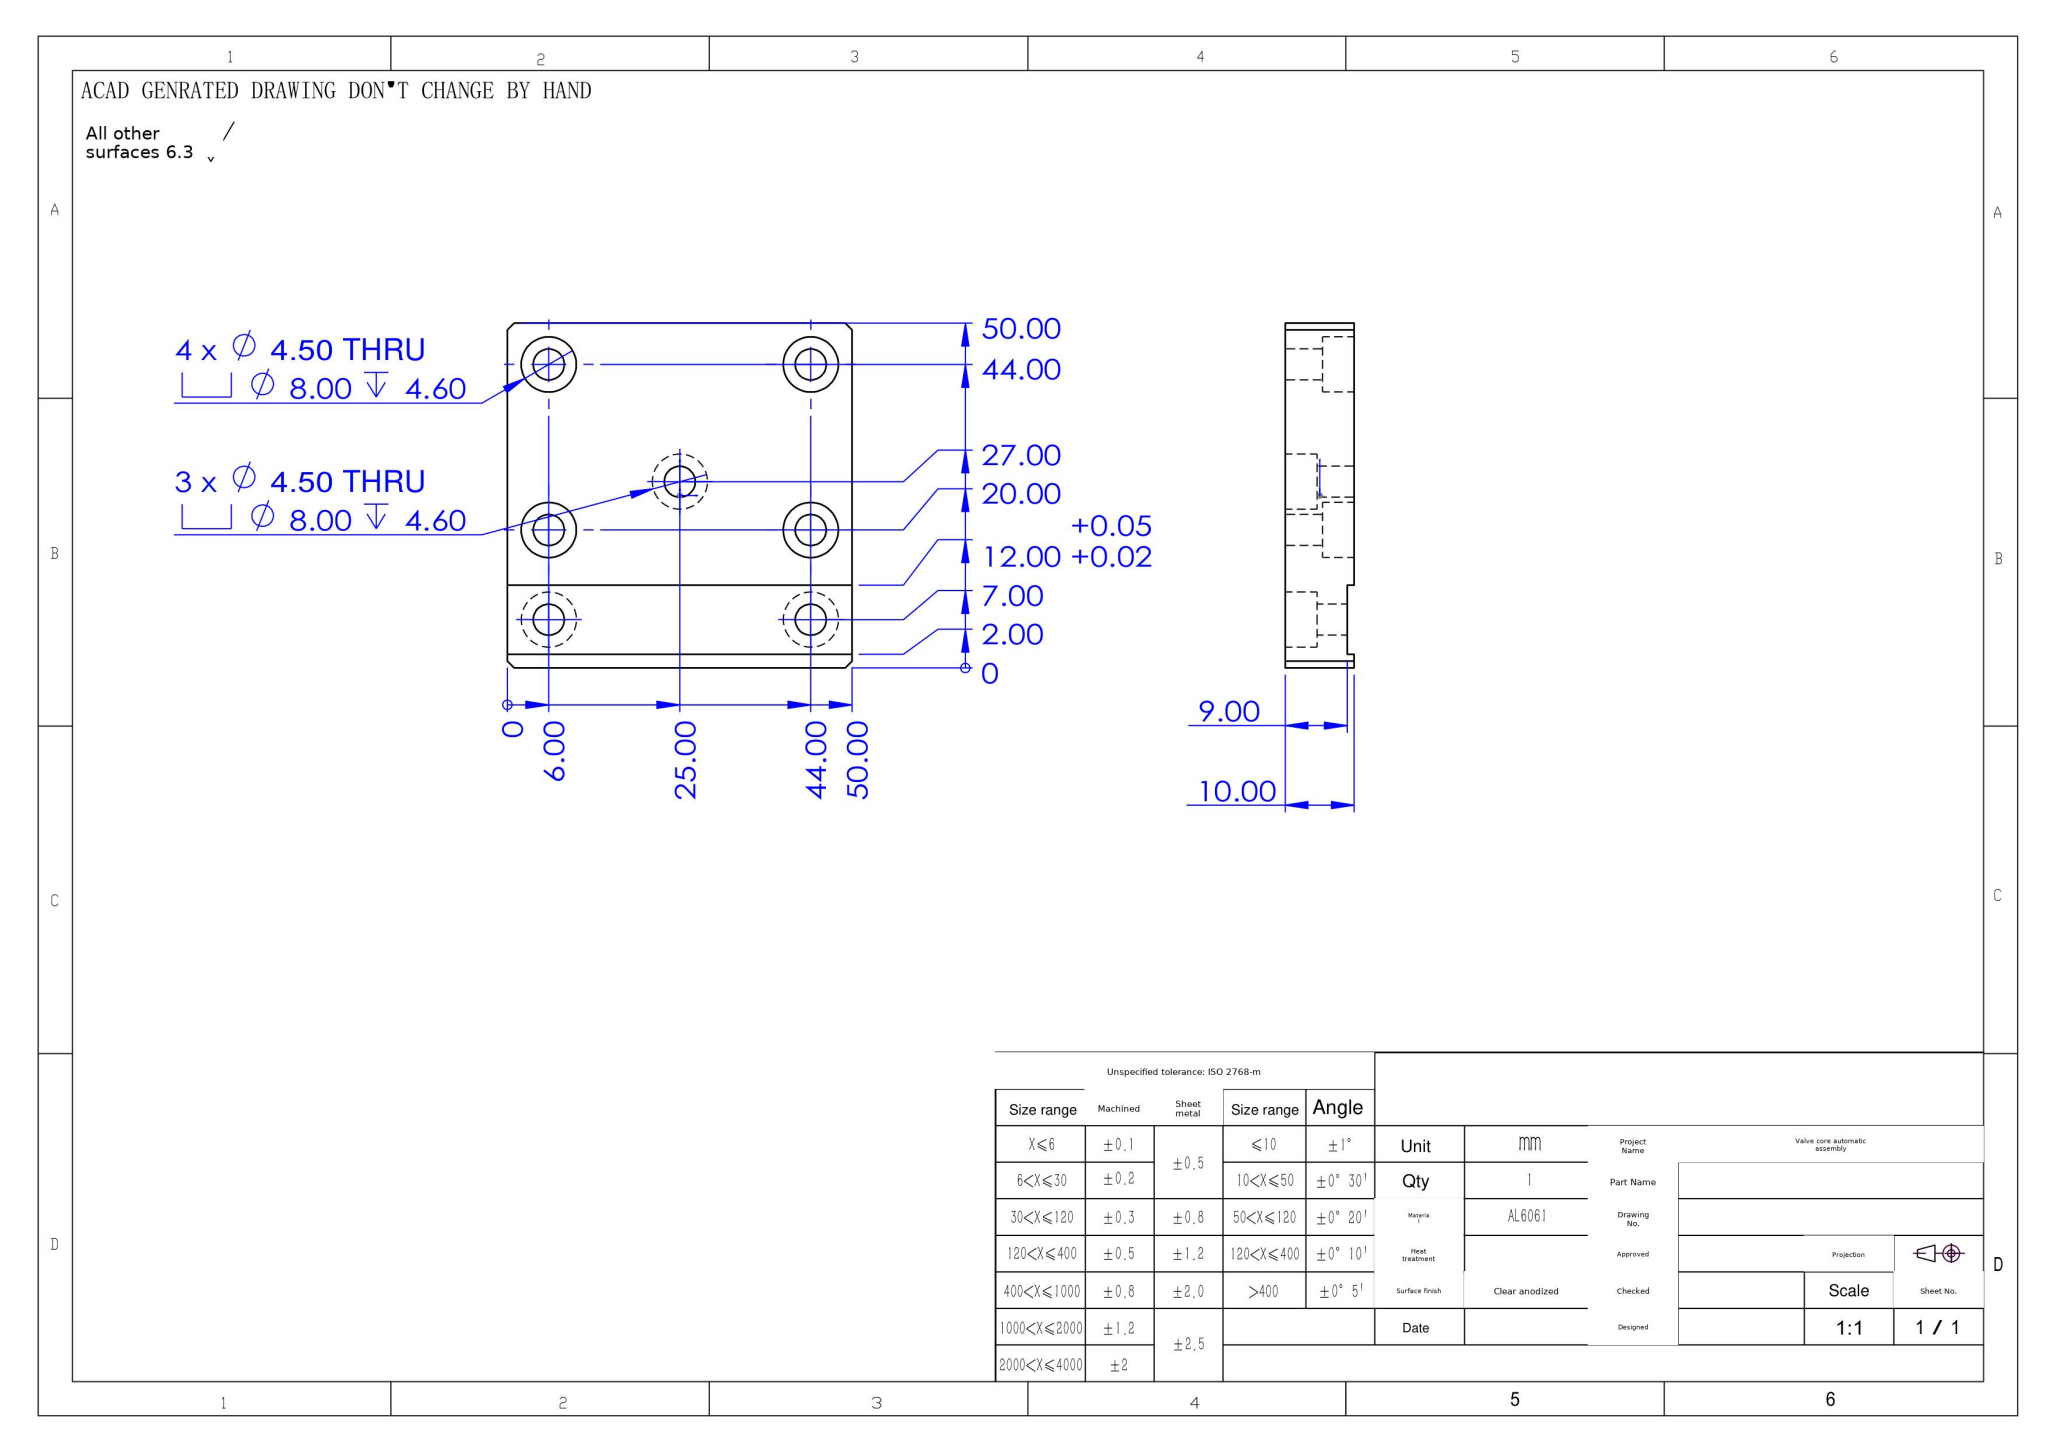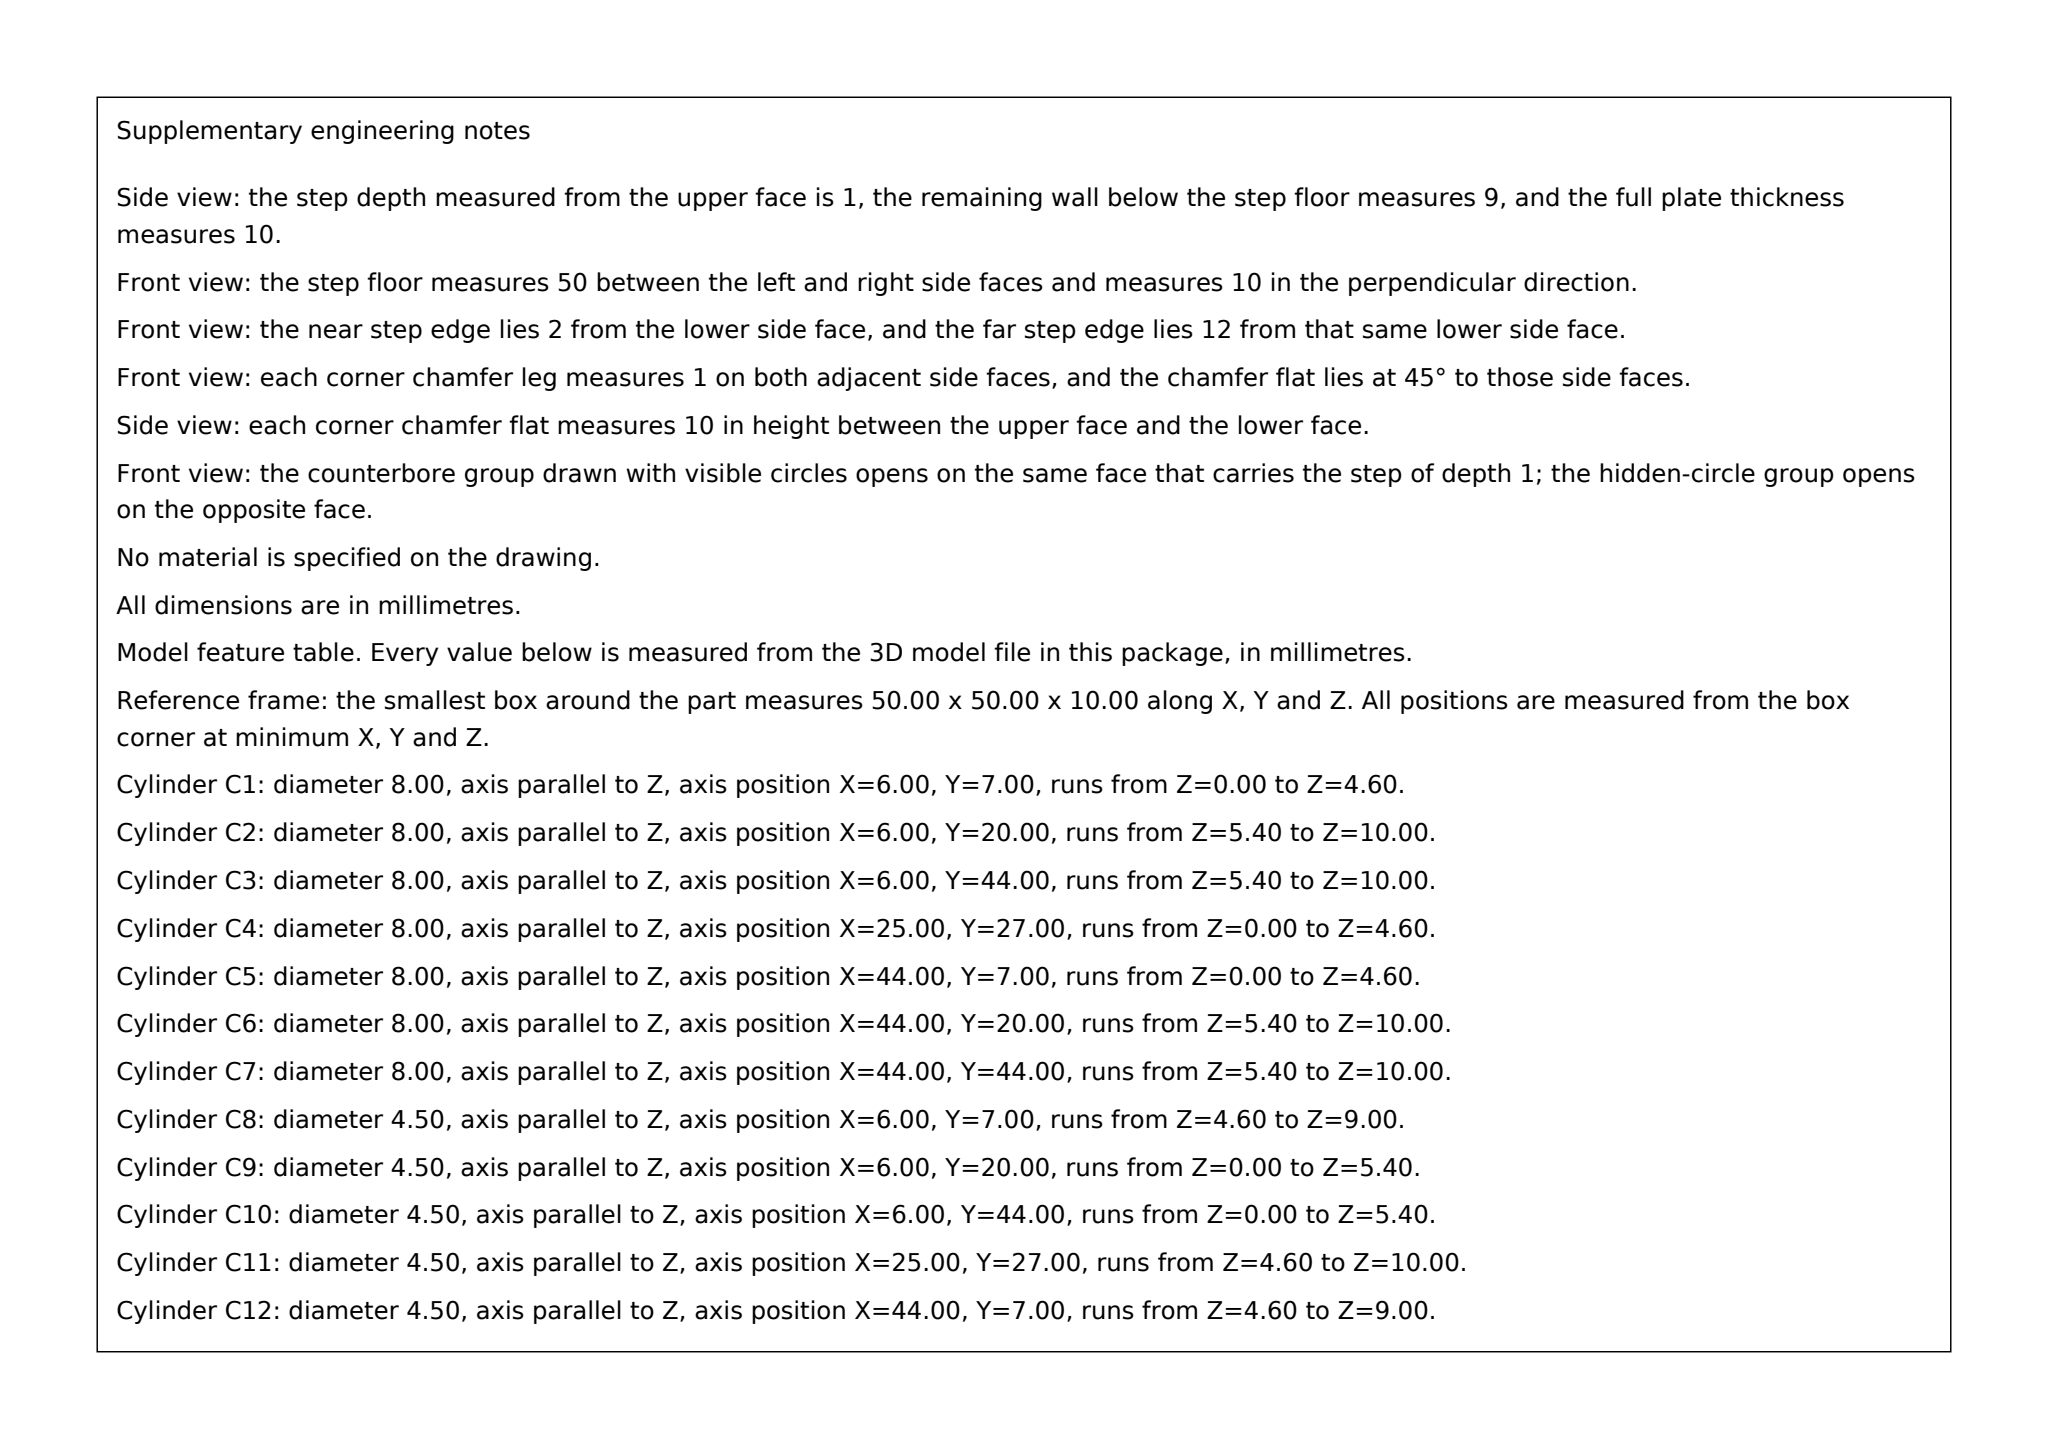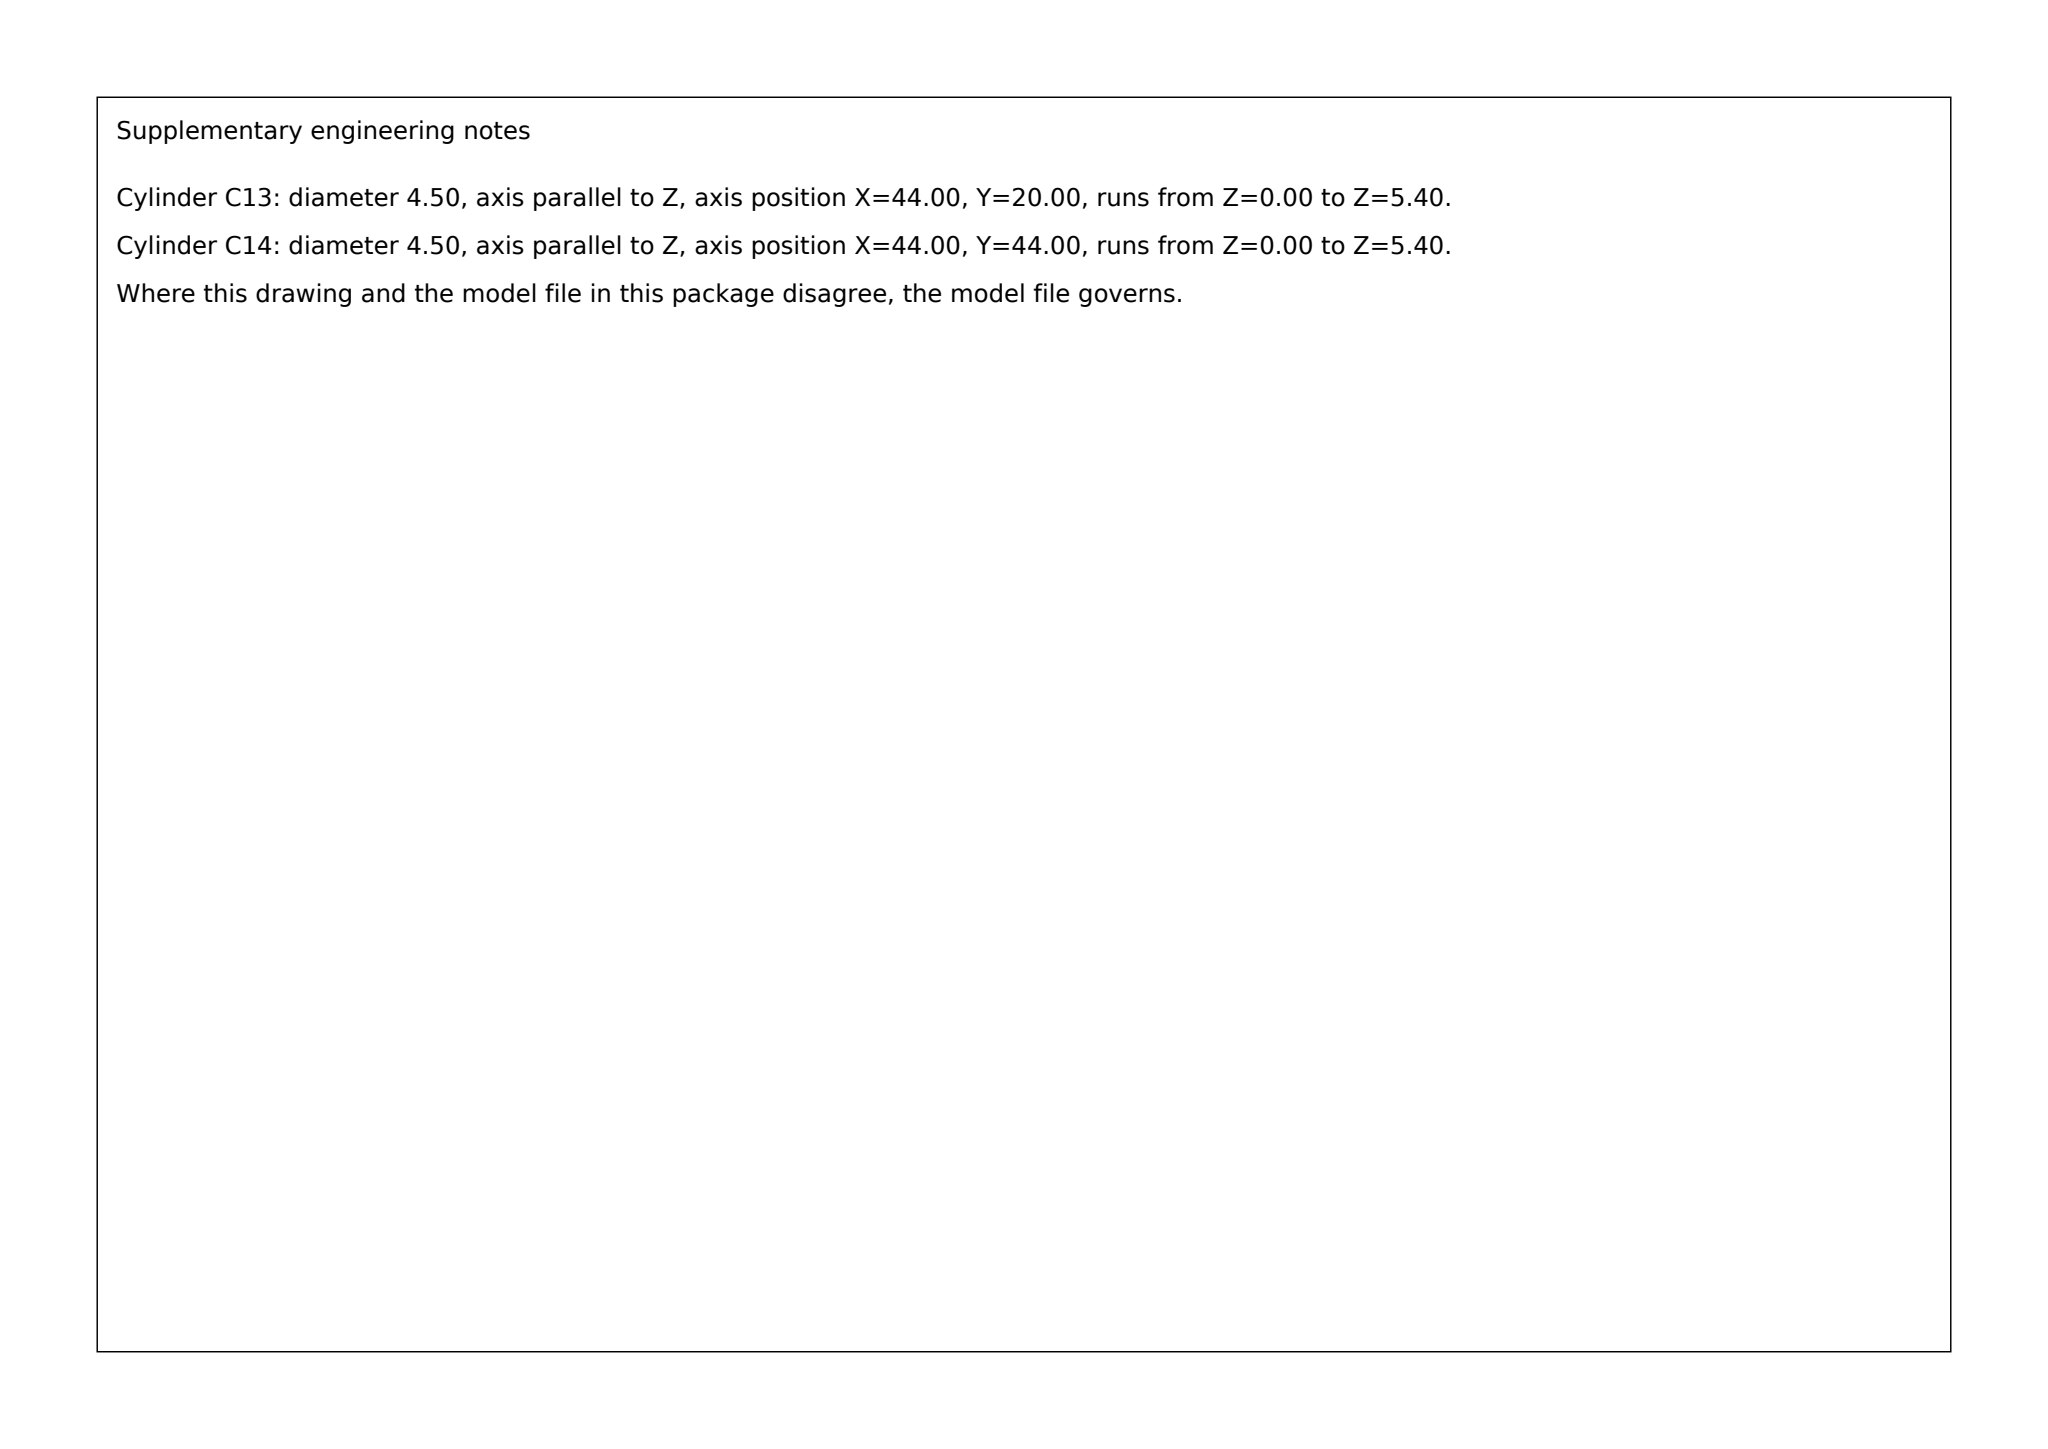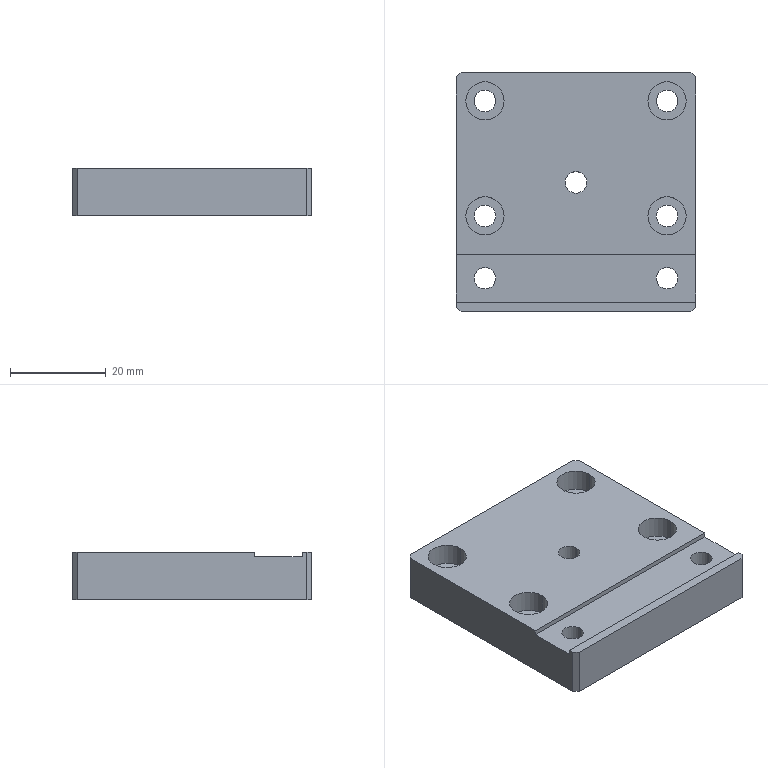Part | SolidWorks | mm | material AL6061 | 1 solid | 49 faces | box 50 x 50 x 10 mm | volume 22292 mm3 | cylinder 28 | plane 21 | commonest cylinder face diameters 8 x14 4.5 x14
Drawing notes:
STEP FACE 12.00 +0.05/+0.02 FROM BOTTOM EDGE (12.02-12.05) | from the solid: Plane normal y at offset 12.0 (x 0-50, z 9-10) bounding the 1 mm deep ledge; measured from y=0 face, datum used by the 2.00/7.00/20.00/27.00/44.00/50.00 vertical chain
build123d program:
from build123d import *

# Parameters (mm, degrees)
SKETCH1_W                                          = 50
SKETCH1_H                                          = 50
BOSS_EXTRUDE1_DEPTH                                = 5
SKETCH2_W                                          = 50
SKETCH2_H                                          = 10
CUT_EXTRUDE1_DEPTH                                 = 1
HOLE_SIZE_ACCORDING_TO_TYPE_1_OF_HEXAG_D           = 4.5
HOLE_SIZE_ACCORDING_TO_TYPE_1_OF_HEXAG_CBORE_D     = 8
HOLE_SIZE_ACCORDING_TO_TYPE_1_OF_HEXAG_CBORE_DEPTH = 4.6
HOLE_SIZE_ACCORDING_TO_TYPE_2_OF_HEXAG_D           = 4.5
HOLE_SIZE_ACCORDING_TO_TYPE_2_OF_HEXAG_CBORE_D     = 8
HOLE_SIZE_ACCORDING_TO_TYPE_2_OF_HEXAG_CBORE_DEPTH = 4.6
CHAMFER1_SIZE                                      = 1


with BuildPart() as part:
    # Sketch1 → Boss-Extrude1 (new, symmetric)
    with BuildSketch(Plane.XY):
        Rectangle(SKETCH1_W, SKETCH1_H)
    extrude(amount=BOSS_EXTRUDE1_DEPTH, both=True)

    # Sketch2 → Cut-Extrude1 (cut)
    with BuildSketch(Plane.XY.offset(5)):
        with Locations((0, -18)):
            Rectangle(SKETCH2_W, SKETCH2_H)
    extrude(amount=-CUT_EXTRUDE1_DEPTH, mode=Mode.SUBTRACT)

    # Hole Size _According to_ Type 1 of Hexag (through all)
    with Locations(Plane(origin=(0, 0, -5), x_dir=(-1, 0, 0), z_dir=(0, 0, -1))):
        with Locations((0, 2), (-19, -18), (19, -18)):
            CounterBoreHole(HOLE_SIZE_ACCORDING_TO_TYPE_1_OF_HEXAG_D / 2, HOLE_SIZE_ACCORDING_TO_TYPE_1_OF_HEXAG_CBORE_D / 2, HOLE_SIZE_ACCORDING_TO_TYPE_1_OF_HEXAG_CBORE_DEPTH)

    # Hole Size _According to_ Type 2 of Hexag (through all)
    with Locations(Plane.XY.offset(5)):
        with Locations((19, 19), (-19, 19), (-19, -5), (19, -5)):
            CounterBoreHole(HOLE_SIZE_ACCORDING_TO_TYPE_2_OF_HEXAG_D / 2, HOLE_SIZE_ACCORDING_TO_TYPE_2_OF_HEXAG_CBORE_D / 2, HOLE_SIZE_ACCORDING_TO_TYPE_2_OF_HEXAG_CBORE_DEPTH)

    # Chamfer1
    chamfer1_edges = [part.edges().sort_by_distance(p)[0] for p in [
        (25, -25, 0),
        (-25, -25, 0),
        (-25, 25, 0),
        (25, 25, 0),
    ]]
    chamfer(chamfer1_edges, length=CHAMFER1_SIZE)


solid = part.part